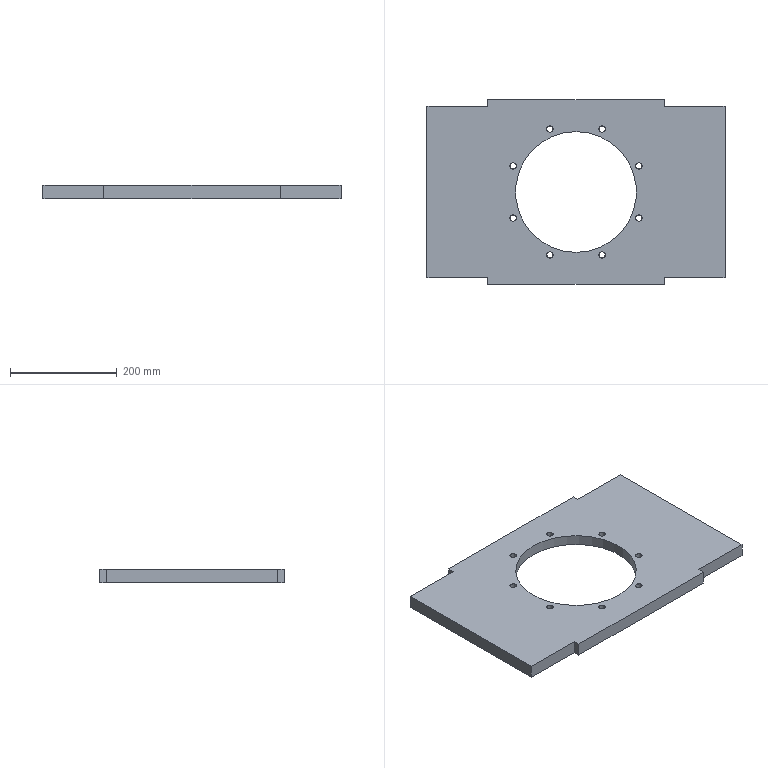Component | NX | CH3404_5-5 | 1 solid | 41 faces | volume 3503584 mm3 | cone 16 | plane 15 | cylinder 10 | commonest cylinder face diameters 11.5 x8 226 x1 300 x1